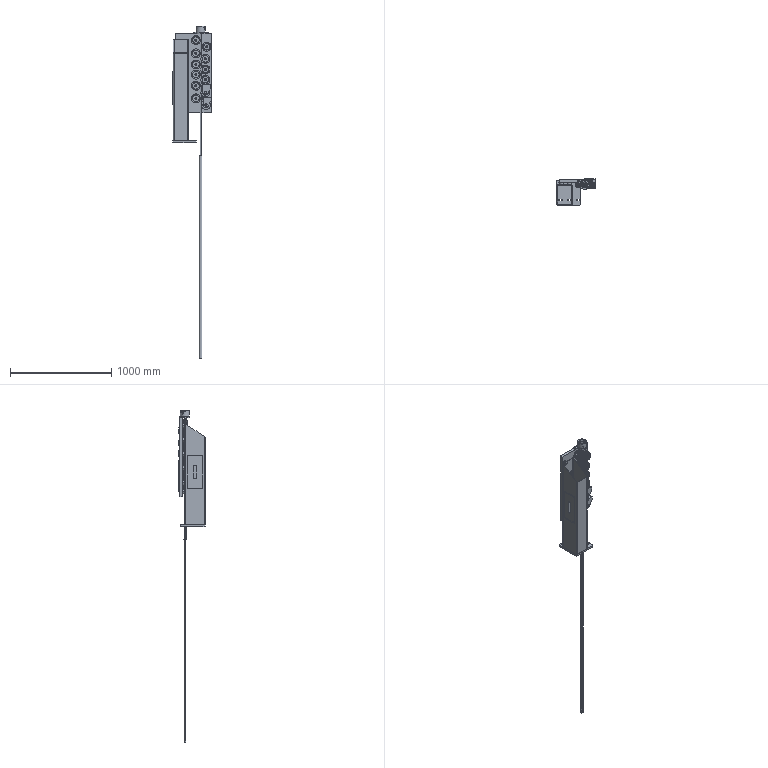Assembly | SolidWorks | mm | 67 component files | 77 solids | 2476 faces | box 382 x 259.1 x 3276.5 mm | volume 16089333 mm3 | cylinder 913 | plane 609 | sphere 352 | cone 324 | torus 278 | commonest cylinder face diameters 8.5 x92 89 x71 35 x64 10 x56 45 x56 11 x48 65 x40 64 x40
Bill of materials:
12AFeedInletPlate | 1 | Q235 | Flat T-shaped plate: a rectangular crossbar with rounded corners joined to a stem that ends in a large semicircular lobe. It has a central cutout made of two overlapping circles and several smaller holes.
12AFeedInletSeat | 1 | Cr12MoV | Thick cylindrical ring with a central bore and one radial slit cut through the wall, plus small cross holes. It resembles a split clamping collar.
12AFeedInletSpacer | 1 | Cr12MoV | Rectangular flat bar or block with two round through-holes, one near each end.
12A10_Steel_Rib | 1 |  | Flat four-lobed outline made of four overlapping circles arranged in a cross, with a tiny gap at the center. In the edge views it shows essentially no thickness.
12AFixedStraighteningWheelCover | 6 | Q235 | Flat circular disc with a small central through-hole. It resembles a plain washer or spacer.
12ASlidingStraighteningWheelPlate | 4 | Q235 | Flat elongated octagonal plate (a rectangle with its four corners chamfered) with two round through-holes side by side.
12ASlidingWheelCover | 4 | Q235 | Flat rectangular plate with two rounded corners at one end and a concave arc cut into the other short end. It has two round through-holes.
12ADoubleGrooveWheel | 10 | GCr15 | Cylindrical wheel with two rounded (semicircular-profile) grooves around its outer surface and a central through-bore. It resembles a double-groove pulley or guide roller.
12ADoubleGrooveWheelAxis | 10 | 45 | Stepped, axially symmetric hub: a thin wide flange with cylindrical bosses of different diameters on each side and a small central hole on one end.
12ADoubleGrooveWheelCover | 10 | 45 | Thin flat circular disc with a central countersunk or conical through-hole and shallow concentric raised steps on one face.
12A6006DeepGrooveBallBearing | 4 | GCr4 | Annular assembly of inner and outer rings with a row of balls between them. It resembles an open radial ball bearing.
12AInnerSideWheel | 2 | Cr12MoV | Short cylindrical sleeve or ring with a thin radial flange at one end and a large central bore. It resembles a flanged bushing.
12AInnerSideWheelAxis | 2 | 40Cr | Axisymmetric stepped part: a thin two-step circular flange between a larger cylindrical boss on one side and a smaller cylindrical boss on the other. The larger boss has a longitudinal slot with a rounded end cut into its open end.
12AOuterSideWheel | 2 | Cr12MoV | Flanged annular sleeve: a short cylindrical sleeve with a thin outer flange at one end, a fillet where the sleeve meets the flange, and a central circular through bore.
12AOuterSideWheelPlate | 2 | Q235 | Flat plate of uniform thickness. One end is rounded and has a single circular through hole. The outline tapers along an angled edge to a wider square end, and that square end has a small rectangular notch across its thickness.
12AOuterSideWheelSeat | 2 | Q235 | Prismatic block with a stepped, roughly T-shaped outline: a wide main body, a narrower extension on one end, and a thin protruding lip or ledge along one long side. The end face of the extension has a groove with a rounded bottom.
12AOuterSideWheelSmallAxis | 2 | 45 | Solid-looking stepped cylindrical plug: a small-diameter nose with a chamfer, a raised collar, a larger main cylinder, and a narrow circumferential groove near the far end.
12ATransverseStraighteningPlate | 1 | Q235 | Rectangular flat plate with a pattern of through cutouts: small round holes, a column of short obround openings with flat sides, a column of wider obround slots, and two thin narrow slots. Small holes are also drilled into the narrow edge faces.
12ATransverseStraighteningSeat | 1 | Q235 | Bracket-like part: a vertical hollow rectangular tube with an obliquely cut top end, joined to a flat base plate. The base plate has rounded corners and six obround slots. A row of small cylindrical studs or bosses runs along one side of the tube.
12ATransverseStraighteningSeatBaffle | 1 | Q235 | Very thin rectangular plate or sheet with rounded corners and one central elongated obround slot running along its long axis.
Mates:
1. concentric | 12ATransverseStraighteningSeat-1 face at (-65.883, 127.46, 486) dir (0, 1, 0) r 5.1 | 12ATransverseStraighteningPlatePart-2/12ATransverseStraighteningPlate-1 face at (-65.883, 127.46, 486) dir (0, -1, 0) r 6.5
2. concentric | 12ATransverseStraighteningSeat-1 face at (8.117, 127.46, 346) dir (0, -1, 0) r 20 | 12ATransverseStraighteningPlatePart-2/12ATransverseStraighteningPlate-1 face at (8.117, 127.46, 346) dir (0, -1, 0) r 6.5
3. coincident | 12ATransverseStraighteningSeat-1 face at (-65.883, 127.46, 486) dir (0, 1, 0) | 12ATransverseStraighteningPlatePart-2/12ATransverseStraighteningPlate-1 face at (87.617, 127.46, 176) dir (0, -1, 0)
4. coincident | 12ATransverseStraighteningPlatePart-2/12ATransverseStraighteningPlate-1 face at (262.617, 127.46, 566) dir (0, 0, 1) | 12AFeedInletPlate-1 face at (159.117, 111.71, 566) dir (0, 0, -1)
5. concentric | 12ATransverseStraighteningPlatePart-2/12ATransverseStraighteningPlate-1 face at (206.617, 141.71, 566) dir (0, 0, 1) r 5.1 | 12AFeedInletPlate-1 sketch segment at (206.617, 141.71, 582) dir (0, 0, 1) r 6.5
6. concentric | 12ATransverseStraighteningPlatePart-2/12ATransverseStraighteningPlate-1 face at (111.617, 141.71, 566) dir (0, 0, 1) r 5.1 | 12AFeedInletPlate-1 sketch segment at (111.617, 141.71, 582) dir (0, 0, 1) r 6.5
7. concentric | 12AFeedInletPlate-1 face at (159.117, 105.71, 566) dir (0, 0, 1) r 44.5 | 12AFeedInletSeat-1 face at (159.117, 105.71, 642) dir (0, 0, -1) r 44.5
8. coincident | 12AFeedInletPlate-1 face at (159.117, 111.71, 582) dir (0, 0, 1) | 12AFeedInletSeat-1 face at (159.117, 105.71, 582) dir (0, 0, -1)
9. concentric | 12AFeedInletSeat-1 face at (211.106, 129.656, 627.5) dir (0.443, 0.8965, 0) r 4.5 | 12AFeedInletSpacer-1 face at (189.508, 85.951, 627.5) dir (-0.443, -0.8965, 0) r 4.5
10. concentric | 12AFeedInletSeat-1 face at (146.557, 161.554, 627.5) dir (0.443, 0.8965, 0) r 4.5 | 12AFeedInletSpacer-1 face at (124.96, 117.849, 627.5) dir (-0.443, -0.8965, 0) r 4.5
11. coincident | 12AFeedInletSeat-1 face at (206.767, 77.422, 612) dir (0.443, 0.8965, 0) | 12AFeedInletSpacer-1 face at (157.234, 101.9, 630) dir (-0.443, -0.8965, 0)
12. coincident | 12ATransverseStraighteningSeat-1 face at (-111.883, -83.04, 509) dir (-1, 0, 0) | 12ATransverseStraighteningSeatBaffle-1 face at (-111.883, 72.21, -119.25) dir (1, 0, 0)
13. width | 12ATransverseStraighteningSeat-1 face at (-101.883, -93.04, 509) dir (0, -1, 0) | 12ATransverseStraighteningSeat-1 face at (28.117, 106.96, 509) dir (0, 1, 0) | 12ATransverseStraighteningSeatBaffle-1 face at (-111.883, 82.21, 181.25) dir (0, 1, 0) | 12ATransverseStraighteningSeatBaffle-1 face at (-111.883, -68.29, 181.25) dir (0, -1, 0)
14. width | 12ATransverseStraighteningSeatBaffle-1 face at (-111.883, 72.21, -129.25) dir (0, 0, -1) | 12ATransverseStraighteningSeatBaffle-1 face at (-111.883, 72.21, 191.25) dir (0, 0, 1) | 12ATransverseStraighteningSeat-1 face at (118.118, 71.96, 181) dir (0, 0, -1) | 12ATransverseStraighteningSeat-1 face at (118.118, 71.96, -119) dir (0, 0, 1)
15. coincident | 12ATransverseStraighteningPlate-1 face at (-44.443, 21.493, 14.25) dir (0, 0, 1) | 12AStraighteningGrooveWheel-29/12ADoubleGrooveWheelAxis-1 face at (-240.943, 3.993, 14.25) dir (0, 0, -1)
16. concentric | 12ATransverseStraighteningPlate-1 face at (-240.943, 46.493, -15.75) dir (0, 0, 1) r 22.5 | 12AStraighteningGrooveWheel-29/12ADoubleGrooveWheelAxis-1 face at (-240.943, 46.493, -14.25) dir (0, 0, -1) r 22.5
17. coincident | 12ATransverseStraighteningPlate-1 face at (-255.085, 63.993, -15.75) dir (0, -1, 0) | 12AStraighteningGrooveWheel-29/12ADoubleGrooveWheelAxis-1 face at (-255.085, 63.993, 42.973) dir (0, 1, 0)
18. coincident | 12ATransverseStraighteningPlate-1 face at (-44.443, 21.493, 14.25) dir (0, 0, 1) | 12AStraighteningGrooveWheel-30/12ADoubleGrooveWheelAxis-1 face at (-130.943, 3.993, 14.25) dir (0, 0, -1)
19. concentric | 12ATransverseStraighteningPlate-1 face at (-130.943, 46.493, -15.75) dir (0, 0, 1) r 22.5 | 12AStraighteningGrooveWheel-30/12ADoubleGrooveWheelAxis-1 face at (-130.943, 46.493, -14.25) dir (0, 0, -1) r 22.5
20. coincident | 12ATransverseStraighteningPlate-1 face at (-145.085, 63.993, -15.75) dir (0, -1, 0) | 12AStraighteningGrooveWheel-30/12ADoubleGrooveWheelAxis-1 face at (-145.085, 63.993, 42.973) dir (0, 1, 0)
21. coincident | 12ATransverseStraighteningPlate-1 face at (-44.443, 21.493, 14.25) dir (0, 0, 1) | 12AStraighteningGrooveWheel-26/12ADoubleGrooveWheelAxis-1 face at (-30.943, 3.993, 14.25) dir (0, 0, -1)
22. concentric | 12ATransverseStraighteningPlate-1 face at (-30.943, 46.493, -15.75) dir (0, 0, 1) r 22.5 | 12AStraighteningGrooveWheel-26/12ADoubleGrooveWheelAxis-1 face at (-30.943, 46.493, -14.25) dir (0, 0, -1) r 22.5
23. coincident | 12ATransverseStraighteningPlate-1 face at (-45.085, 63.993, -15.75) dir (0, -1, 0) | 12AStraighteningGrooveWheel-26/12ADoubleGrooveWheelAxis-1 face at (-45.085, 63.993, 42.973) dir (0, 1, 0)
24. coincident | 12ATransverseStraighteningPlate-1 face at (-44.443, 21.493, 14.25) dir (0, 0, 1) | 12AStraighteningGrooveWheel-31/12ADoubleGrooveWheelAxis-1 face at (79.057, 3.993, 14.25) dir (0, 0, -1)
25. concentric | 12ATransverseStraighteningPlate-1 face at (79.057, 46.493, -15.75) dir (0, 0, 1) r 22.5 | 12AStraighteningGrooveWheel-31/12ADoubleGrooveWheelAxis-1 face at (79.057, 46.493, -14.25) dir (0, 0, -1) r 22.5
26. coincident | 12ATransverseStraighteningPlate-1 face at (64.915, 63.993, -15.75) dir (0, -1, 0) | 12AStraighteningGrooveWheel-31/12ADoubleGrooveWheelAxis-1 face at (64.915, 63.993, 42.973) dir (0, 1, 0)
27. coincident | 12ATransverseStraighteningPlate-1 face at (-44.443, 21.493, 14.25) dir (0, 0, 1) | 12AStraighteningGrooveWheel-27/12ADoubleGrooveWheelAxis-1 face at (204.057, 3.993, 14.25) dir (0, 0, -1)
28. concentric | 12ATransverseStraighteningPlate-1 face at (204.057, 46.493, -15.75) dir (0, 0, 1) r 22.5 | 12AStraighteningGrooveWheel-27/12ADoubleGrooveWheelAxis-1 face at (204.057, 46.493, -14.25) dir (0, 0, -1) r 22.5
29. coincident | 12ATransverseStraighteningPlate-1 face at (189.915, 63.993, -15.75) dir (0, -1, 0) | 12AStraighteningGrooveWheel-27/12ADoubleGrooveWheelAxis-1 face at (189.915, 63.993, 42.973) dir (0, 1, 0)
30. coincident | 12ATransverseStraighteningPlate-1 face at (-44.443, 21.493, 14.25) dir (0, 0, 1) | 12AStraighteningGrooveWheel-28/12ADoubleGrooveWheelAxis-1 face at (-263.943, 153.993, 14.25) dir (0, 0, -1)
31. coincident | 12ATransverseStraighteningPlate-1 face at (-323.943, 168.135, -14.25) dir (1, 0, 0) | 12AStraighteningGrooveWheel-28/12ADoubleGrooveWheelAxis-1 face at (-323.943, 139.851, 42.973) dir (-1, 0, 0)
32. coincident | 12ATransverseStraighteningPlate-1 face at (-44.443, 21.493, 14.25) dir (0, 0, 1) | 12AStraighteningGrooveWheel-32/12ADoubleGrooveWheelAxis-1 face at (-143.943, 139.993, 14.25) dir (0, 0, -1)
33. coincident | 12ATransverseStraighteningPlate-1 face at (-203.943, 168.135, -14.25) dir (1, 0, 0) | 12AStraighteningGrooveWheel-32/12ADoubleGrooveWheelAxis-1 face at (-203.943, 125.851, 42.973) dir (-1, 0, 0)
34. coincident | 12ATransverseStraighteningPlate-1 face at (-44.443, 21.493, 14.25) dir (0, 0, 1) | 12AStraighteningGrooveWheel-23/12ADoubleGrooveWheelAxis-1 face at (-38.943, 139.993, 14.25) dir (0, 0, -1)
35. coincident | 12ATransverseStraighteningPlate-1 face at (-98.943, 168.135, -14.25) dir (1, 0, 0) | 12AStraighteningGrooveWheel-23/12ADoubleGrooveWheelAxis-1 face at (-98.943, 125.851, 42.973) dir (-1, 0, 0)
36. coincident | 12ATransverseStraighteningPlate-1 face at (-44.443, 21.493, 14.25) dir (0, 0, 1) | 12AStraighteningGrooveWheel-25/12ADoubleGrooveWheelAxis-1 face at (61.057, 139.993, 14.25) dir (0, 0, -1)
37. coincident | 12ATransverseStraighteningPlate-1 face at (1.057, 168.135, -14.25) dir (1, 0, 0) | 12AStraighteningGrooveWheel-25/12ADoubleGrooveWheelAxis-1 face at (1.057, 125.851, 42.973) dir (-1, 0, 0)
38. coincident | 12ATransverseStraighteningPlate-1 face at (164.057, 169.485, -14.25) dir (-1, 0, 0) | 12AStraighteningInnerWheel-3/12AInnerSideWheelAxis-2 face at (164.057, 170.438, 77.467) dir (1, 0, 0)
39. coincident | 12ATransverseStraighteningPlate-1 face at (-44.443, 21.493, 14.25) dir (0, 0, 1) | 12AStraighteningInnerWheel-3/12AInnerSideWheelAxis-2 face at (143.557, 175.993, 14.25) dir (0, 0, -1)
40. coincident | 12ATransverseStraighteningPlate-1 face at (289.057, 169.485, -14.25) dir (-1, 0, 0) | 12AStraighteningInnerWheel-2/12AInnerSideWheelAxis-2 face at (289.057, 175.06, 77.467) dir (1, 0, 0)
41. coincident | 12ATransverseStraighteningPlate-1 face at (-44.443, 21.493, 14.25) dir (0, 0, 1) | 12AStraighteningInnerWheel-2/12AInnerSideWheelAxis-2 face at (268.557, 180.615, 14.25) dir (0, 0, -1)
42. coincident | 12ATransverseStraighteningPlate-1 face at (-44.443, 21.493, 14.25) dir (0, 0, 1) | 12AStraighteningOuterWheel-3/12AOuterSideWheelSeat-1 face at (98.557, 114.993, 14.25) dir (0, 0, -1)
43. coincident | 12ATransverseStraighteningPlate-1 face at (74.557, 180.993, -14.25) dir (1, 0, 0) | 12AStraighteningOuterWheel-3/12AOuterSideWheelSeat-1 face at (74.557, 129.993, -14.35) dir (-1, 0, 0)
44. coincident | 12ATransverseStraighteningPlate-1 face at (199.557, 180.993, -14.25) dir (1, 0, 0) | 12AStraighteningOuterWheel-2/12AOuterSideWheelSeat-1 face at (199.557, 133.582, -14.35) dir (-1, 0, 0)
45. coincident | 12ATransverseStraighteningPlate-1 face at (-44.443, 21.493, 14.25) dir (0, 0, 1) | 12AStraighteningOuterWheel-2/12AOuterSideWheelSeat-1 face at (223.557, 118.582, 14.25) dir (0, 0, -1)
46. coincident | 12ATransverseStraighteningPlate-1 face at (-44.443, 21.493, -14.25) dir (0, 0, -1) | 12ASlidingStraighteningWheelPlate-7 face at (-306.443, 153.993, -14.25) dir (0, 0, 1)
47. concentric | 12AStraighteningGrooveWheel-28/12ADoubleGrooveWheelAxis-1 face at (-306.443, 138.993, -14.25) dir (0, 0, -1) r 4.25 | 12ASlidingStraighteningWheelPlate-7 face at (-306.443, 138.993, -14.25) dir (0, 0, 1) r 5.5
48. concentric | 12AStraighteningGrooveWheel-28/12ADoubleGrooveWheelAxis-1 face at (-306.443, 168.993, -14.25) dir (0, 0, -1) r 4.25 | 12ASlidingStraighteningWheelPlate-7 face at (-306.443, 168.993, -14.25) dir (0, 0, 1) r 5.5
49. coincident | 12ATransverseStraighteningPlate-1 face at (-44.443, 21.493, -14.25) dir (0, 0, -1) | 12ASlidingStraighteningWheelPlate-8 face at (-186.443, 139.993, -14.25) dir (0, 0, 1)
50. concentric | 12AStraighteningGrooveWheel-32/12ADoubleGrooveWheelAxis-1 face at (-186.443, 124.993, -14.25) dir (0, 0, -1) r 4.25 | 12ASlidingStraighteningWheelPlate-8 face at (-186.443, 124.993, -14.25) dir (0, 0, 1) r 5.5
51. concentric | 12AStraighteningGrooveWheel-32/12ADoubleGrooveWheelAxis-1 face at (-186.443, 154.993, -14.25) dir (0, 0, -1) r 4.25 | 12ASlidingStraighteningWheelPlate-8 face at (-186.443, 154.993, -14.25) dir (0, 0, 1) r 5.5
52. coincident | 12ATransverseStraighteningPlate-1 face at (-44.443, 21.493, -14.25) dir (0, 0, -1) | 12ASlidingStraighteningWheelPlate-9 face at (-81.443, 139.993, -14.25) dir (0, 0, 1)
53. concentric | 12AStraighteningGrooveWheel-23/12ADoubleGrooveWheelAxis-1 face at (-81.443, 124.993, -14.25) dir (0, 0, -1) r 4.25 | 12ASlidingStraighteningWheelPlate-9 face at (-81.443, 124.993, -14.25) dir (0, 0, 1) r 5.5
54. concentric | 12AStraighteningGrooveWheel-23/12ADoubleGrooveWheelAxis-1 face at (-81.443, 154.993, -14.25) dir (0, 0, -1) r 4.25 | 12ASlidingStraighteningWheelPlate-9 face at (-81.443, 154.993, -14.25) dir (0, 0, 1) r 5.5
55. coincident | 12ATransverseStraighteningPlate-1 face at (-44.443, 21.493, -14.25) dir (0, 0, -1) | 12ASlidingStraighteningWheelPlate-10 face at (18.557, 139.993, -14.25) dir (0, 0, 1)
56. concentric | 12AStraighteningGrooveWheel-25/12ADoubleGrooveWheelAxis-1 face at (18.557, 124.993, -14.25) dir (0, 0, -1) r 4.25 | 12ASlidingStraighteningWheelPlate-10 face at (18.557, 124.993, -14.25) dir (0, 0, 1) r 5.5
57. concentric | 12AStraighteningGrooveWheel-25/12ADoubleGrooveWheelAxis-1 face at (18.557, 154.993, -14.25) dir (0, 0, -1) r 4.25 | 12ASlidingStraighteningWheelPlate-10 face at (18.557, 154.993, -14.25) dir (0, 0, 1) r 5.5
58. coincident | 12AStraighteningGrooveWheel-29/12ADoubleGrooveWheelAxis-1 face at (-240.943, 24.993, -14.25) dir (0, 0, -1) | 12AFixedStraighteningWheelCover-11 face at (-240.943, 46.493, -14.25) dir (0, 0, 1)
59. concentric | 12AStraighteningGrooveWheel-29/12ADoubleGrooveWheelAxis-1 face at (-240.943, 46.493, -14.25) dir (0, 0, -1) r 4.25 | 12AFixedStraighteningWheelCover-11 face at (-240.943, 46.493, -14.25) dir (0, 0, -1) r 5.5
60. coincident | 12AStraighteningGrooveWheel-30/12ADoubleGrooveWheelAxis-1 face at (-130.943, 24.993, -14.25) dir (0, 0, -1) | 12AFixedStraighteningWheelCover-12 face at (-130.943, 46.493, -14.25) dir (0, 0, 1)
61. concentric | 12AStraighteningGrooveWheel-30/12ADoubleGrooveWheelAxis-1 face at (-130.943, 46.493, -14.25) dir (0, 0, -1) r 4.25 | 12AFixedStraighteningWheelCover-12 face at (-130.943, 46.493, -14.25) dir (0, 0, -1) r 5.5
62. coincident | 12AStraighteningGrooveWheel-26/12ADoubleGrooveWheelAxis-1 face at (-30.943, 24.993, -14.25) dir (0, 0, -1) | 12AFixedStraighteningWheelCover-13 face at (-30.943, 46.493, -14.25) dir (0, 0, 1)
63. concentric | 12AStraighteningGrooveWheel-26/12ADoubleGrooveWheelAxis-1 face at (-30.943, 46.493, -14.25) dir (0, 0, -1) r 4.25 | 12AFixedStraighteningWheelCover-13 face at (-30.943, 46.493, -14.25) dir (0, 0, -1) r 5.5
64. coincident | 12AStraighteningGrooveWheel-31/12ADoubleGrooveWheelAxis-1 face at (79.057, 24.993, -14.25) dir (0, 0, -1) | 12AFixedStraighteningWheelCover-14 face at (79.057, 46.493, -14.25) dir (0, 0, 1)
65. concentric | 12AStraighteningGrooveWheel-31/12ADoubleGrooveWheelAxis-1 face at (79.057, 46.493, -14.25) dir (0, 0, -1) r 4.25 | 12AFixedStraighteningWheelCover-14 face at (79.057, 46.493, -14.25) dir (0, 0, -1) r 5.5
66. coincident | 12AStraighteningGrooveWheel-27/12ADoubleGrooveWheelAxis-1 face at (204.057, 24.993, -14.25) dir (0, 0, -1) | 12AFixedStraighteningWheelCover-10 face at (204.057, 46.493, -14.25) dir (0, 0, 1)
67. concentric | 12AStraighteningGrooveWheel-27/12ADoubleGrooveWheelAxis-1 face at (204.057, 46.493, -14.25) dir (0, 0, -1) r 4.25 | 12AFixedStraighteningWheelCover-10 face at (204.057, 46.493, -14.25) dir (0, 0, -1) r 5.5
68. coincident | 12ATransverseStraighteningPlate-1 face at (-44.443, 21.493, -14.25) dir (0, 0, -1) | 12ASlidingWheelCover-12 face at (268.557, 137.115, -14.25) dir (0, 0, 1)
69. concentric | 12AStraighteningInnerWheel-2/12AInnerSideWheelAxis-2 face at (268.557, 147.115, -14.25) dir (0, 0, -1) r 5.1 | 12ASlidingWheelCover-12 face at (268.557, 147.115, -14.25) dir (0, 0, -1) r 6.5
70. concentric | 12AStraighteningInnerWheel-2/12AInnerSideWheelAxis-2 face at (268.557, 127.115, -14.25) dir (0, 0, -1) r 5.1 | 12ASlidingWheelCover-12 face at (268.557, 127.115, -14.25) dir (0, 0, -1) r 6.5
71. coincident | 12ATransverseStraighteningPlate-1 face at (-44.443, 21.493, -14.25) dir (0, 0, -1) | 12ASlidingWheelCover-10 face at (143.557, 132.493, -14.25) dir (0, 0, 1)
72. concentric | 12AStraighteningInnerWheel-3/12AInnerSideWheelAxis-2 face at (143.557, 142.493, -14.25) dir (0, 0, -1) r 5.1 | 12ASlidingWheelCover-10 face at (143.557, 142.493, -14.25) dir (0, 0, -1) r 6.5
73. concentric | 12AStraighteningInnerWheel-3/12AInnerSideWheelAxis-2 face at (143.557, 122.493, -14.25) dir (0, 0, -1) r 5.1 | 12ASlidingWheelCover-10 face at (143.557, 122.493, -14.25) dir (0, 0, -1) r 6.5
74. coincident | 12AStraighteningOuterWheel-3/12AOuterSideWheelSeat-1 face at (83.557, 129.993, -14.35) dir (0, 0, -1) | 12ASlidingWheelCover-9 face at (83.557, 139.993, -14.35) dir (0, 0, 1)
75. concentric | 12AStraighteningOuterWheel-3/12AOuterSideWheelSeat-1 face at (83.557, 129.993, -14.35) dir (0, 0, -1) r 4.25 | 12ASlidingWheelCover-9 face at (83.557, 129.993, -14.35) dir (0, 0, -1) r 6.5
76. concentric | 12AStraighteningOuterWheel-3/12AOuterSideWheelSeat-1 face at (83.557, 149.993, -14.35) dir (0, 0, -1) r 4.25 | 12ASlidingWheelCover-9 face at (83.557, 149.993, -14.35) dir (0, 0, -1) r 6.5
77. coincident | 12AStraighteningOuterWheel-2/12AOuterSideWheelSeat-1 face at (208.557, 133.582, -14.35) dir (0, 0, -1) | 12ASlidingWheelCover-11 face at (208.557, 143.582, -14.35) dir (0, 0, 1)
78. concentric | 12AStraighteningOuterWheel-2/12AOuterSideWheelSeat-1 face at (208.557, 133.582, -14.35) dir (0, 0, -1) r 4.25 | 12ASlidingWheelCover-11 face at (208.557, 133.582, -14.35) dir (0, 0, -1) r 6.5
79. concentric | 12AStraighteningOuterWheel-2/12AOuterSideWheelSeat-1 face at (208.557, 153.582, -14.35) dir (0, 0, -1) r 4.25 | 12ASlidingWheelCover-11 face at (208.557, 153.582, -14.35) dir (0, 0, -1) r 6.5
80. concentric | 12ATransverseStraighteningPlate-1 face at (-370.943, 46.493, -15.75) dir (0, 0, 1) r 22.5 | 12AStraighteningGrooveWheel-33/12ADoubleGrooveWheelAxis-1 face at (-370.943, 46.493, -14.25) dir (0, 0, -1) r 22.5
81. coincident | 12ATransverseStraighteningPlate-1 face at (-385.085, 63.993, -15.75) dir (0, -1, 0) | 12AStraighteningGrooveWheel-33/12ADoubleGrooveWheelAxis-1 face at (-385.085, 63.993, 42.973) dir (0, 1, 0)
82. coincident | 12ATransverseStraighteningPlate-1 face at (-44.443, 21.493, 14.25) dir (0, 0, 1) | 12AStraighteningGrooveWheel-33/12ADoubleGrooveWheelAxis-1 face at (-370.943, 3.993, 14.25) dir (0, 0, -1)
83. concentric | 12AStraighteningOuterWheel-3/12AOuterSideWheel-3 face at (143.557, 139.993, 56.25) dir (0, 0, 1) r 40 | 12AStraighteningInnerWheel-3/12AInnerSideWheel-2 face at (143.557, 139.993, 36.75) dir (0, 0, 1) r 40
84. distance | 12A10_Steel_Rib-1 plane at (-434.443, 93.243, 29.25) dir (0, 0, 1) | 12ATransverseStraighteningPlate-1 face at (-44.443, 21.493, 14.25) dir (0, 0, 1)
85. distance | 12A10_Steel_Rib-1 plane at (-434.443, 93.243, 29.25) dir (0, 1, 0) | 12ATransverseStraighteningPlate-1 face at (-434.443, -153.507, 14.25) dir (0, -1, 0)
86. concentric | 12AStraighteningGrooveWheel-28/12ADoubleGrooveWheelAxis-1 face at (-306.443, 153.993, -14.25) dir (0, 0, -1) r 22.5 | 12ATransverseStraighteningPlate-1 face at (-306.443, 153.993, -14.25) dir (0, 0, 1) r 22.5
87. coincident | 12ATransverseStraighteningPlate-1 face at (-434.443, 196.493, 14.25) dir (-1, 0, 0) | 12A10_Steel_Rib-1 face at (-434.443, 93.243, 29.25) dir (-1, 0, 0)
88. distance | 12AStraighteningGrooveWheel-32/12ADoubleGrooveWheelAxis-1 face at (-186.443, 139.993, -14.25) dir (0, 0, -1) r 22.5 | 12ATransverseStraighteningPlate-1 face at (-434.443, -153.507, 14.25) dir (0, -1, 0)
89. distance | 12AStraighteningGrooveWheel-23/12ADoubleGrooveWheelAxis-1 face at (-81.443, 139.993, -14.25) dir (0, 0, -1) r 22.5 | 12ATransverseStraighteningPlate-1 face at (-434.443, -153.507, 14.25) dir (0, -1, 0)
90. distance | 12AStraighteningGrooveWheel-25/12ADoubleGrooveWheelAxis-1 face at (18.557, 139.993, -14.25) dir (0, 0, -1) r 22.5 | 12ATransverseStraighteningPlate-1 face at (-434.443, -153.507, 14.25) dir (0, -1, 0)
91. distance | 12AStraighteningInnerWheel-3/12AInnerSideWheel-2 face at (143.557, 139.993, 36.75) dir (0, 0, 1) r 40 | 12ATransverseStraighteningPlate-1 face at (-434.443, -153.507, 14.25) dir (0, -1, 0)
92. concentric | 12ADoubleGrooveWheel-1 face at (-21.086, 27.564, 0) dir (-1, 0, 0) r 17.5 | 12ADoubleGrooveWheelAxis-1 face at (-53.086, 27.564, 0) dir (-1, 0, 0) r 17.5
93. coincident | 12ADoubleGrooveWheel-1 face at (-17.086, 60.064, 0) dir (-1, 0, 0) | 12ADoubleGrooveWheelAxis-1 face at (-17.086, 37.457, 14.436) dir (1, 0, 0)
94. concentric | 12ADoubleGrooveWheel-1 face at (-21.086, 27.564, 0) dir (-1, 0, 0) r 17.5 | 12ADoubleGrooveWheelCover-1 face at (10.414, 27.564, 0) dir (-1, 0, 0) r 32
95. coincident | 12ADoubleGrooveWheel-1 face at (12.914, 45.064, 0) dir (1, 0, 0) | 12ADoubleGrooveWheelCover-1 face at (12.914, 12.617, 9.101) dir (-1, 0, 0)
96. concentric | 12AInnerSideWheelAxis-2 face at (37.315, 22.195, 0) dir (1, 0, 0) r 15 | 12A6006DeepGrooveBallBearing-1 face at (-17.105, 22.195, 0) dir (-1, 0, 0) r 15
97. coincident | 12AInnerSideWheel-2 face at (-11.185, 22.55, 27.498) dir (1, 0, 0) | 12A6006DeepGrooveBallBearing-1 face at (-11.185, 41.508, 18.145) dir (-1, 0, 0)
98. concentric | 12AInnerSideWheel-2 face at (-13.685, 22.195, 0) dir (-1, 0, 0) r 40 | 12A6006DeepGrooveBallBearing-1 face at (-4.685, 22.195, 0) dir (-1, 0, 0) r 27.5
99. coincident | 12AInnerSideWheelAxis-2 face at (1.815, 37.195, 0) dir (-1, 0, 0) | 12A6006DeepGrooveBallBearing-1 face at (1.815, 36.188, 13.147) dir (1, 0, 0)
100. coincident | 12AOuterSideWheelSeat-1 face at (-104.984, 52.669, 15) dir (0, 1, 0) | 12AOuterSideWheelPlate-1 face at (-79.984, 52.669, 60) dir (0, -1, 0)
101. coincident | 12AOuterSideWheelSeat-1 face at (-104.984, 52.669, 15) dir (-1, 0, 0) | 12AOuterSideWheelPlate-1 face at (-104.984, 52.669, -15) dir (-1, 0, 0)
102. coincident | 12AOuterSideWheelSeat-1 face at (-104.984, 56.669, -4) dir (0, 0, -1) | 12AOuterSideWheelPlate-1 face at (-104.984, 56.669, -4) dir (0, 0, 1)
103. concentric | 12AOuterSideWheelPlate-1 face at (-79.984, 52.669, 60) dir (0, 1, 0) r 12.5 | 12AOuterSideWheelSmallAxis-1 face at (-79.984, 52.669, 60) dir (0, 1, 0) r 12.5
104. coincident | 12AOuterSideWheelPlate-1 face at (-79.984, 52.669, 60) dir (0, -1, 0) | 12AOuterSideWheelSmallAxis-1 face at (-79.984, 52.669, 60) dir (0, 1, 0)
105. concentric | 12AOuterSideWheelSmallAxis-1 face at (-79.984, 31.669, 60) dir (0, 1, 0) r 15 | 12A6006DeepGrooveBallBearing-1 face at (-79.984, 29.748, 60) dir (0, -1, 0) r 15
106. coincident | 12AOuterSideWheelSmallAxis-1 edge at (-79.984, 48.669, 60) dir (0, -1, 0) r 17.5 | 12A6006DeepGrooveBallBearing-1 face at (-64.767, 48.669, 48.291) dir (0, 1, 0)
107. coincident | 12AOuterSideWheel-3 face at (-107.208, 35.669, 56.116) dir (0, 1, 0) | 12A6006DeepGrooveBallBearing-1 face at (-58.982, 35.669, 43.839) dir (0, -1, 0)
108. concentric | 12AOuterSideWheel-3 face at (-79.984, 48.669, 60) dir (0, 1, 0) r 27.5 | 12A6006DeepGrooveBallBearing-1 face at (-79.984, 42.169, 60) dir (0, -1, 0) r 27.5